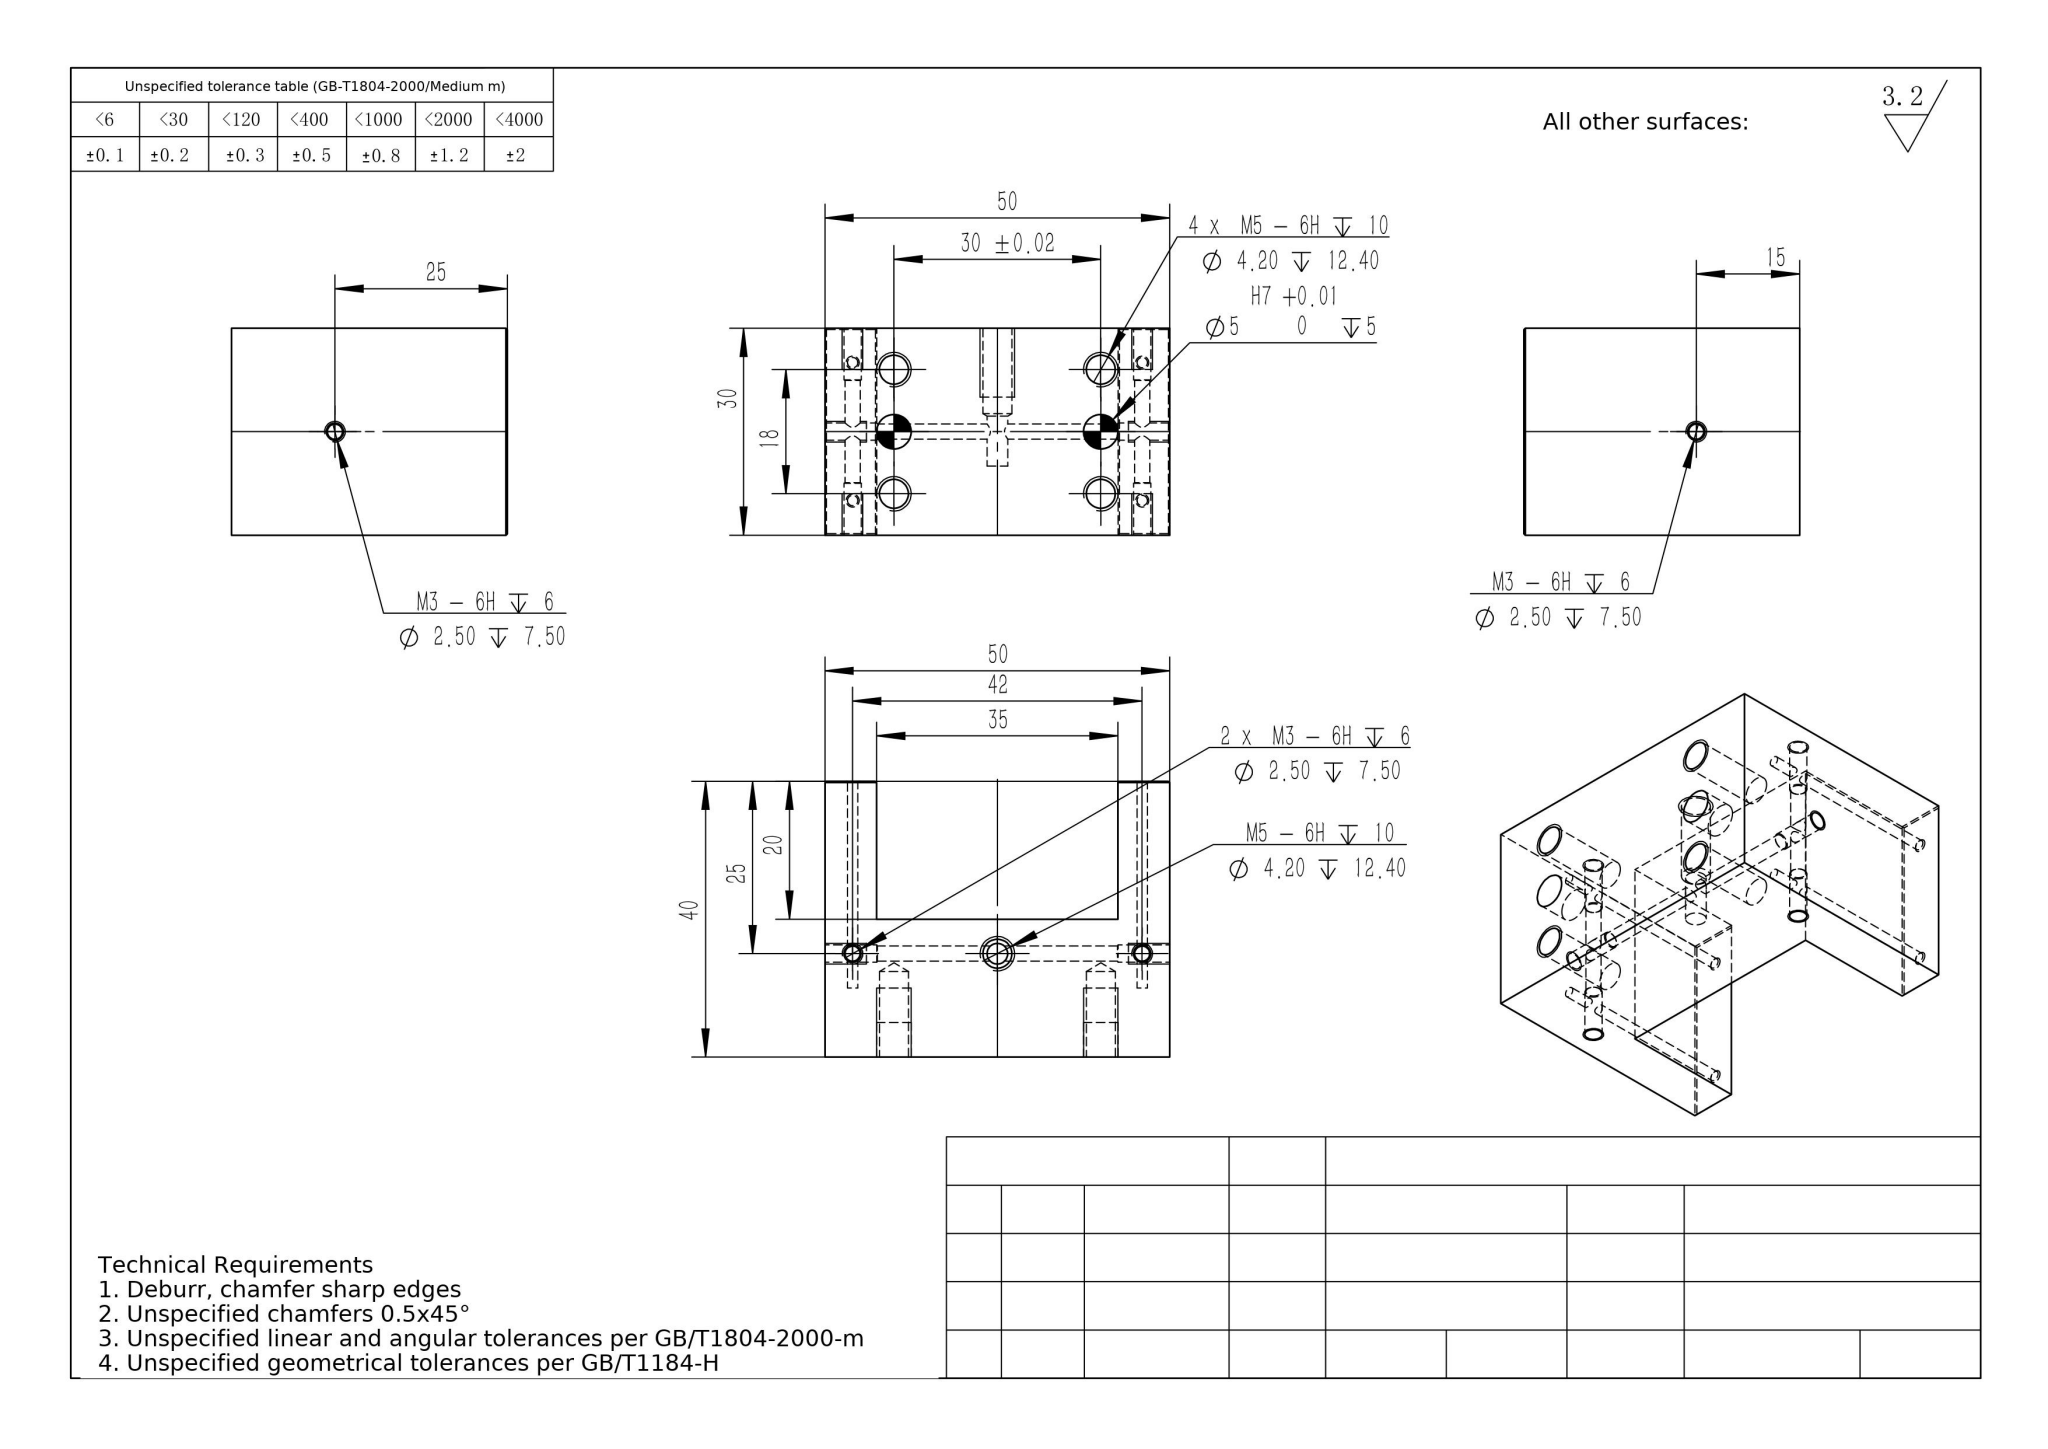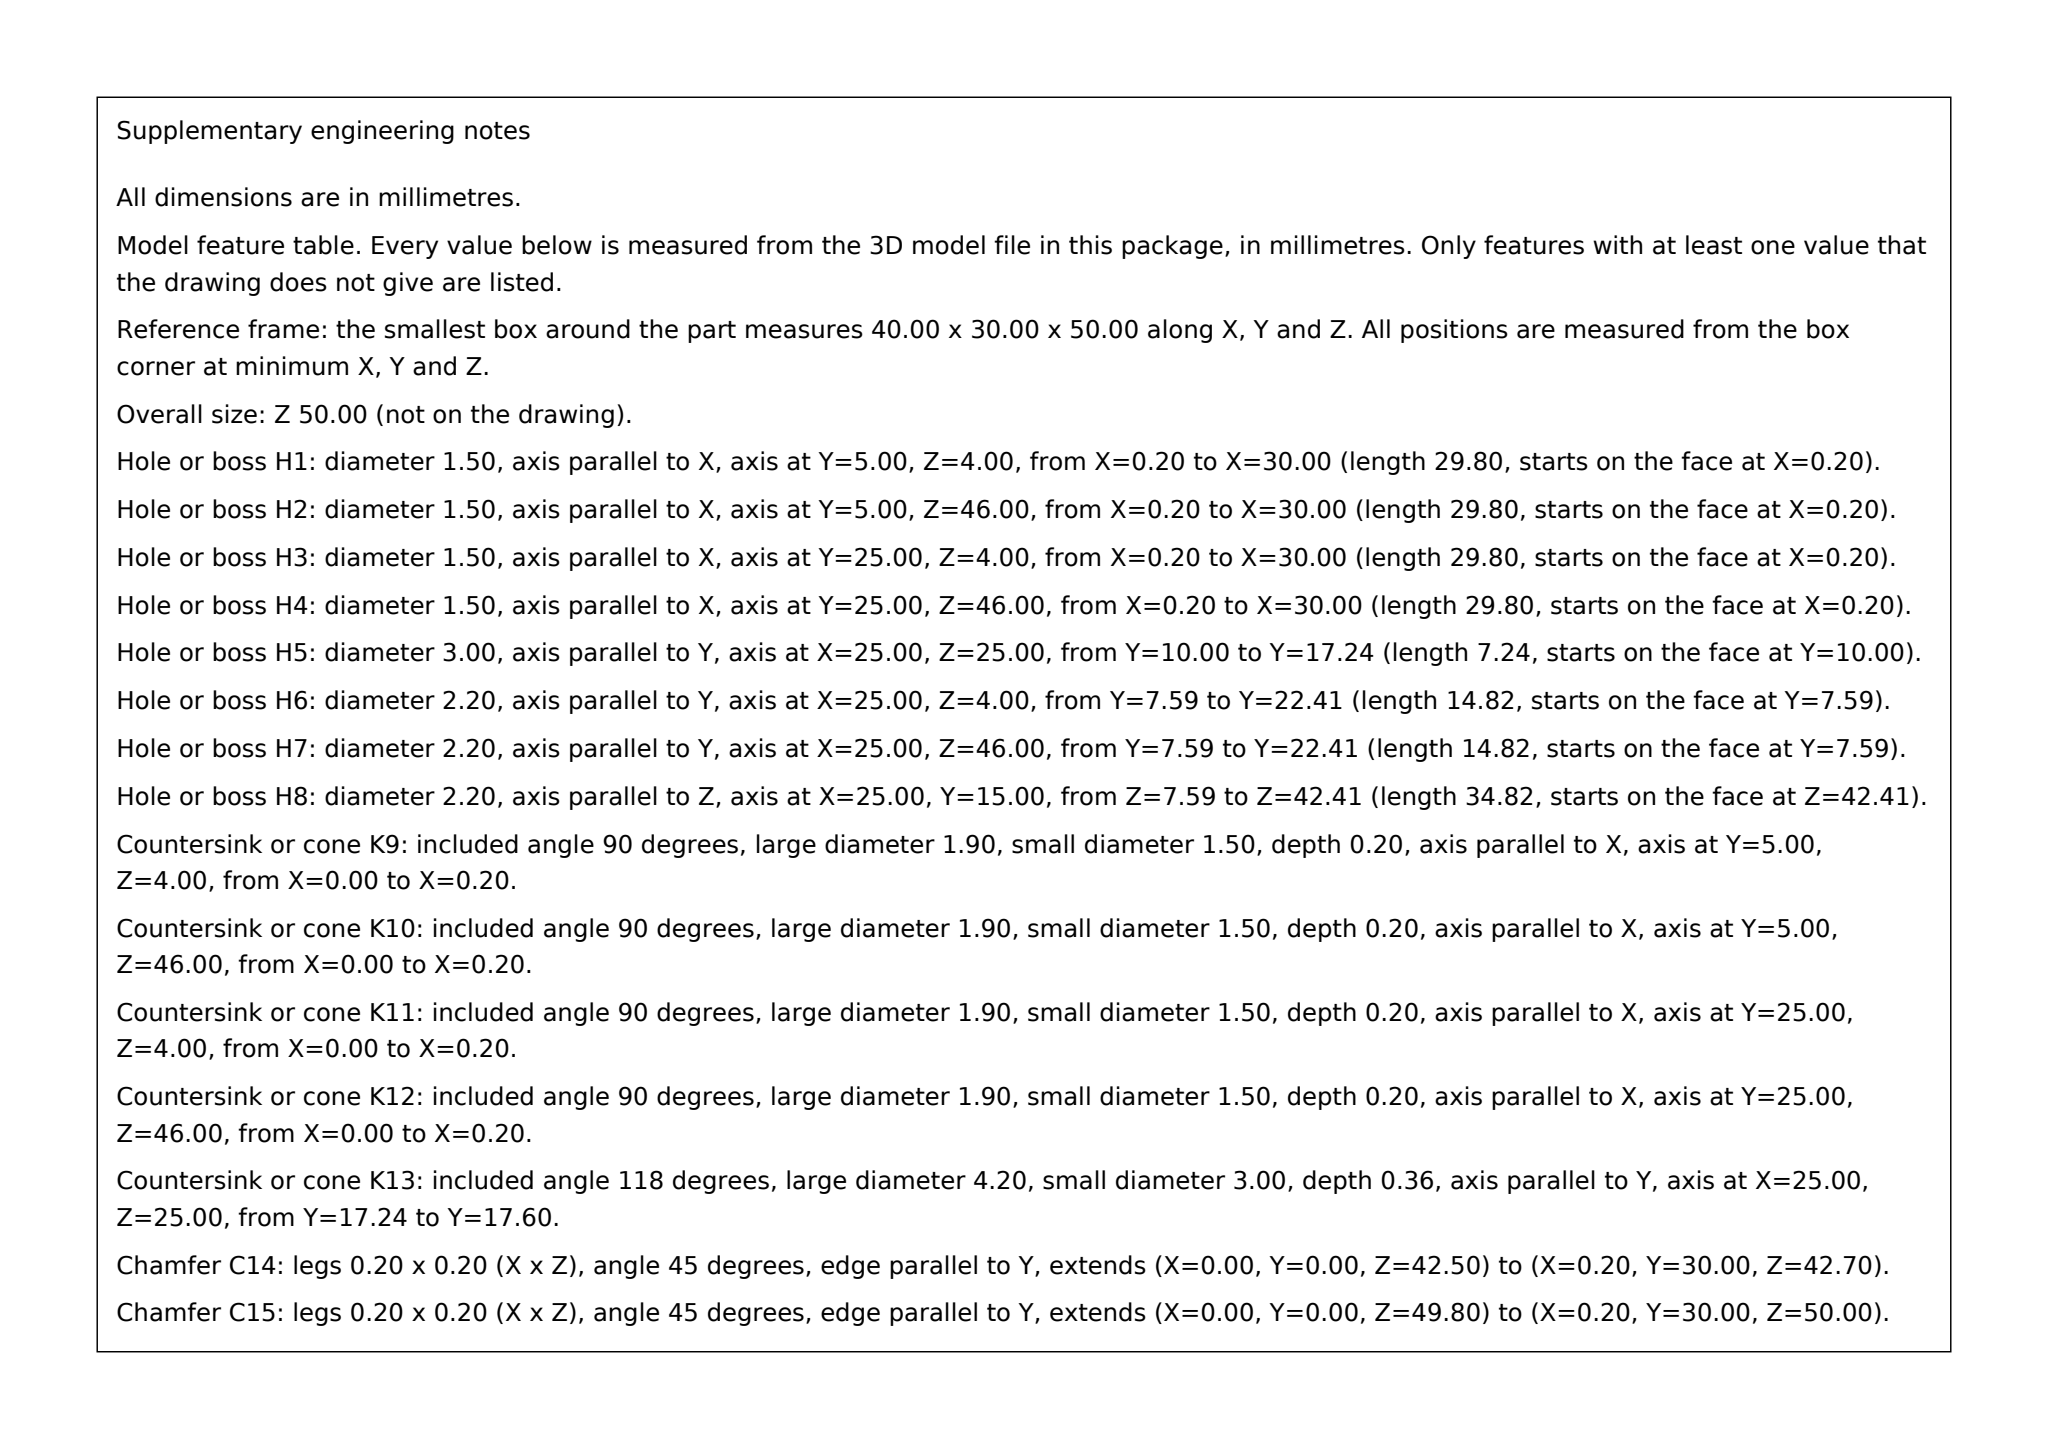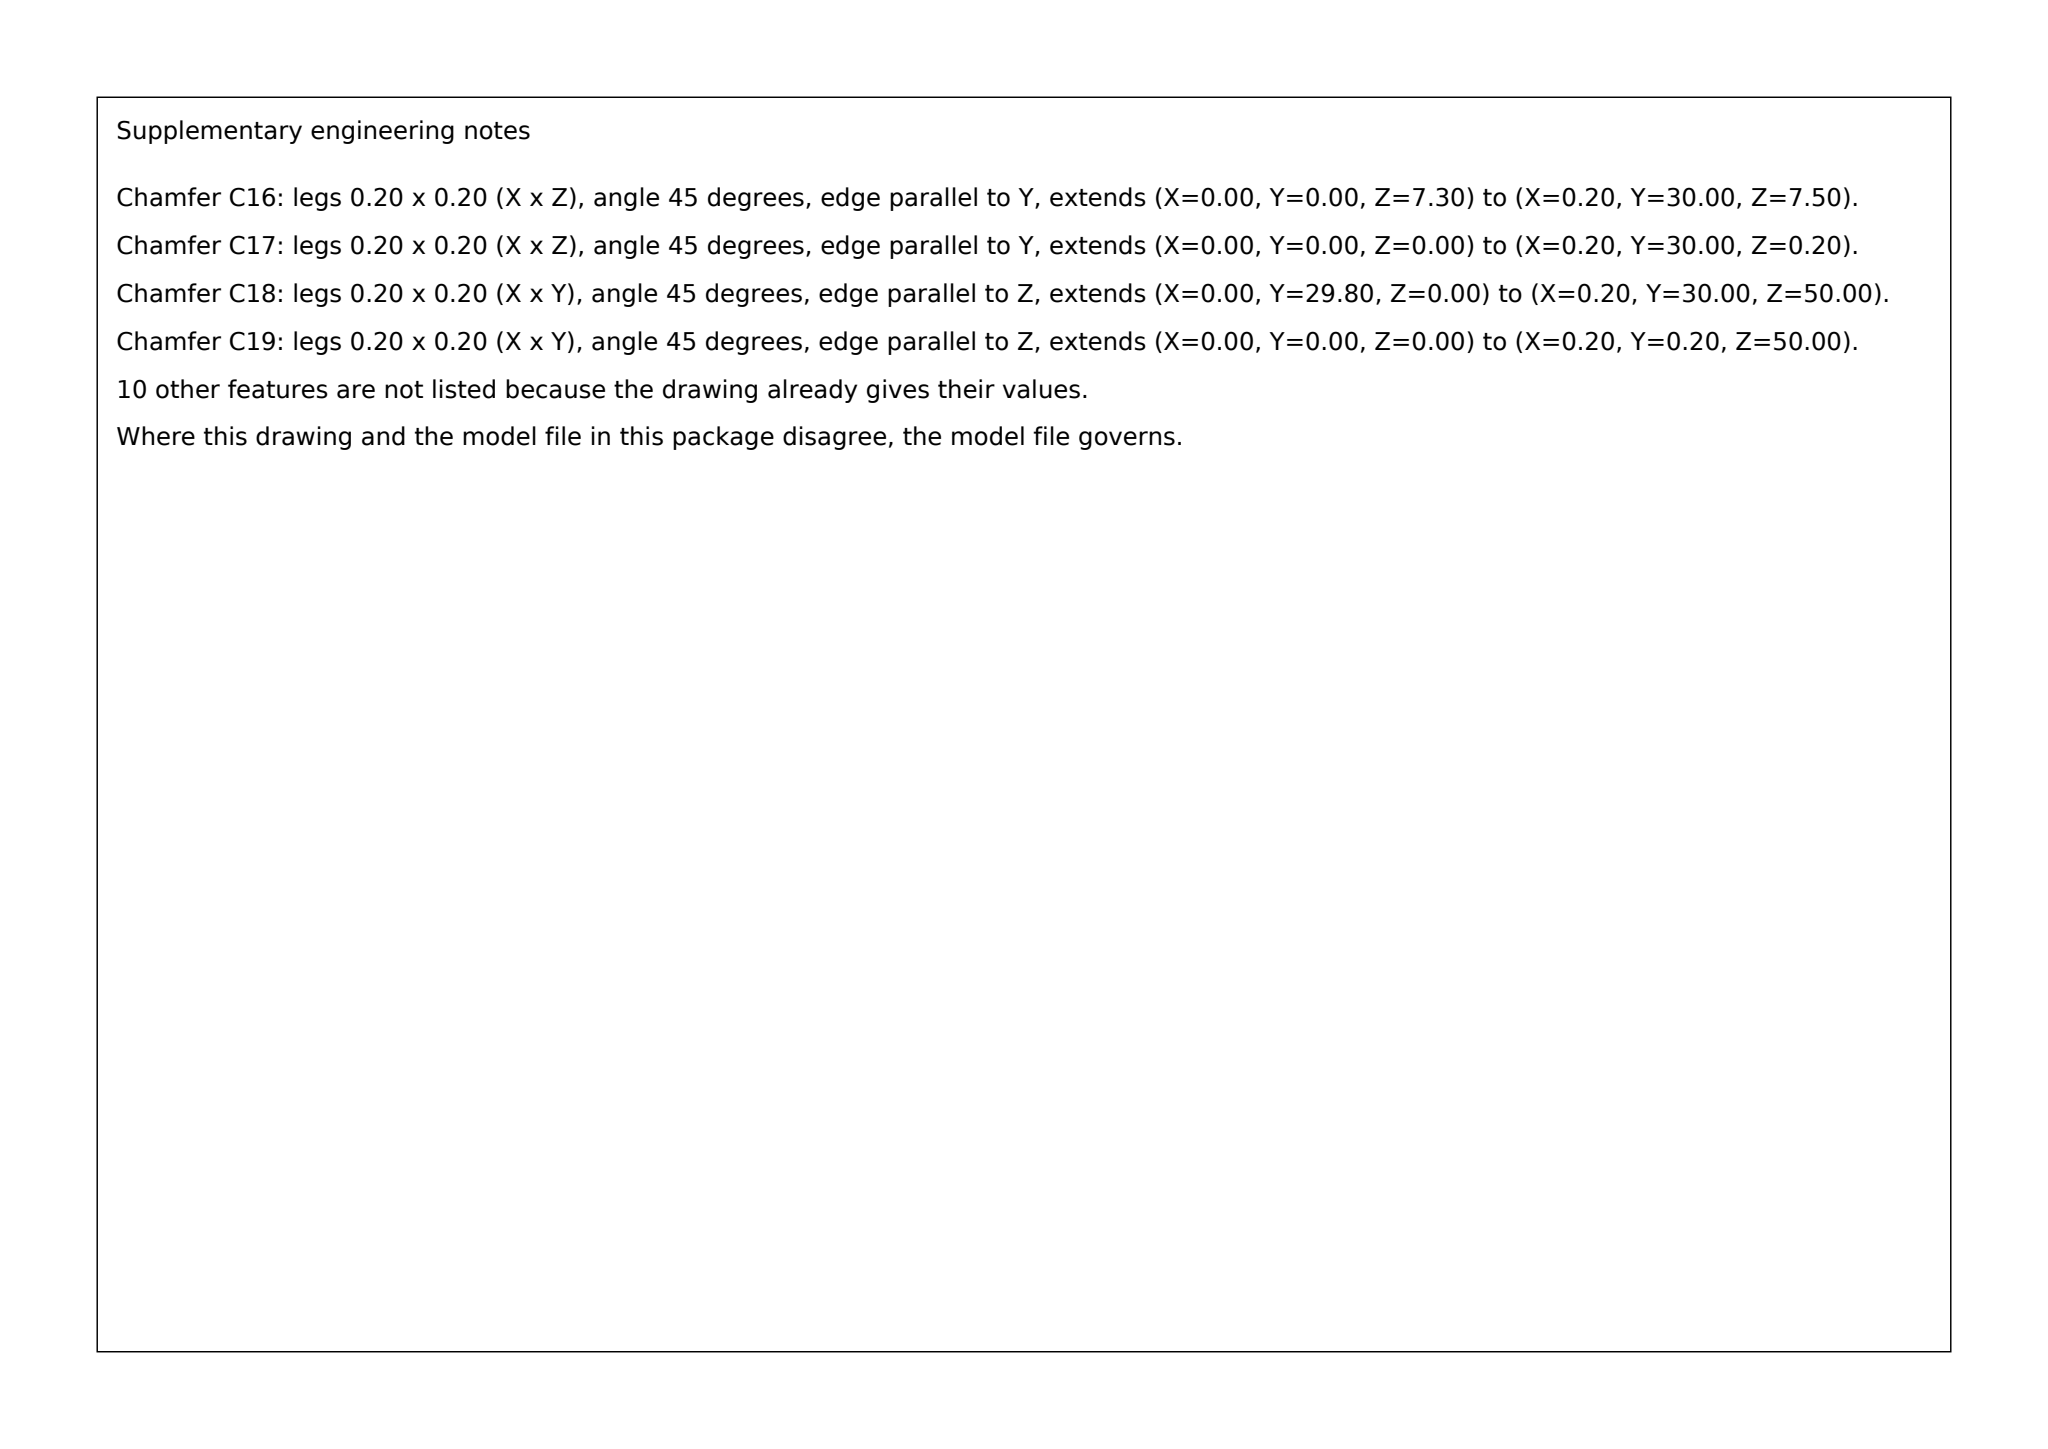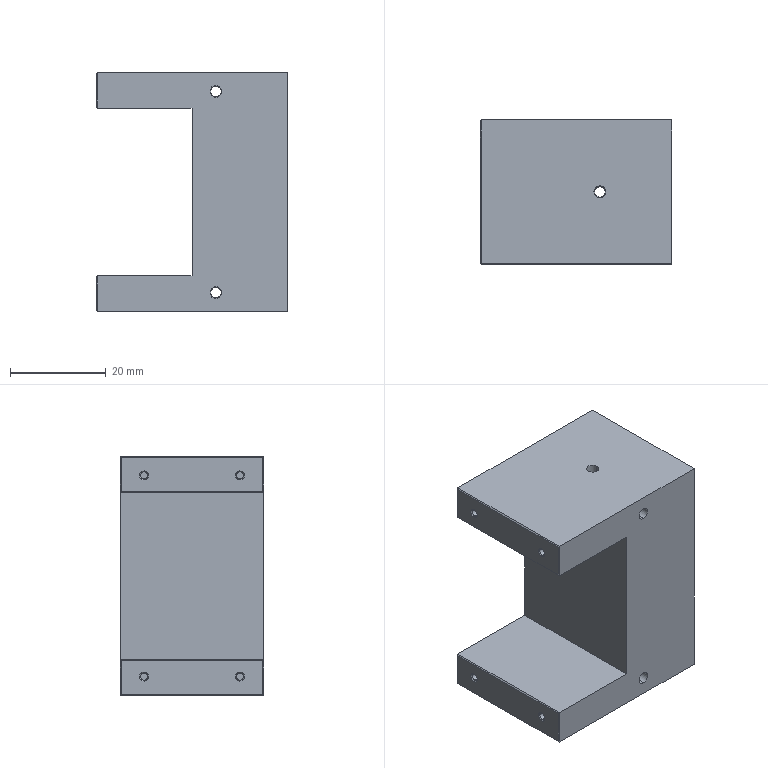Part | SolidWorks | mm | 1 solid | 111 faces | box 40 x 30 x 50 mm | volume 37227 mm3 | cylinder 56 | cone 30 | plane 25 | commonest cylinder face diameters 1.5 x16 2.5 x12 2.2 x12 4.2 x10 5 x4 3 x2
build123d program:
from build123d import *

# Parameters (mm, degrees)
SKETCH1_W             = 50
SKETCH1_H             = 30
BOSS_EXTRUDE1_DEPTH   = 40
SKETCH2_R             = 0.75
CUT_EXTRUDE1_DEPTH    = 30
SKETCH3_R             = 1.1
CUT_EXTRUDE2_DEPTH    = 56.902
SKETCH4_R             = 1.1
CUT_EXTRUDE3_DEPTH    = 66.765
SKETCH5_W             = 20
SKETCH5_H             = 35
CUT_EXTRUDE4_DEPTH    = 56.902
SKETCH6_R             = 1.5
CUT_EXTRUDE5_DEPTH    = 20
M3_TAPPED_HOLE3_D     = 2.5
M3_TAPPED_HOLE3_DEPTH = 7.5
M3_TAPPED_HOLE3_TIP   = 0.7511
M3_TAPPED_HOLE4_D     = 2.5
M3_TAPPED_HOLE4_DEPTH = 7.5
M3_TAPPED_HOLE4_TIP   = 0.7511
M3_TAPPED_HOLE2_D     = 2.5
M3_TAPPED_HOLE2_DEPTH = 7.5
M3_TAPPED_HOLE2_TIP   = 0.7511
M3_TAPPED_HOLE1_D     = 2.5
M3_TAPPED_HOLE1_DEPTH = 7.5
M3_TAPPED_HOLE1_TIP   = 0.7511
M5_TAPPED_HOLE5_D     = 4.2
M5_TAPPED_HOLE5_DEPTH = 12.4
M5_TAPPED_HOLE5_TIP   = 1.262
M5_TAPPED_HOLE6_D     = 4.2
M5_TAPPED_HOLE6_DEPTH = 12.4
M5_TAPPED_HOLE6_TIP   = 1.262
SKETCH20_R            = 2.5
CUT_EXTRUDE6_DEPTH    = 5
CHAMFER1_SIZE         = 0.2


with BuildPart() as part:
    # Sketch1 → Boss-Extrude1 (new body)
    with BuildSketch(Plane(origin=(0, 0, 0), x_dir=(0, 0, -1), z_dir=(1, 0, 0))):
        Rectangle(SKETCH1_W, SKETCH1_H)
    extrude(amount=BOSS_EXTRUDE1_DEPTH)

    # Sketch2 → Cut-Extrude1 (cut)
    with BuildSketch(Plane.ZY):
        with Locations((-21, 10)):
            Circle(SKETCH2_R)
        with Locations(Location((-21, -10, 0), (0, 0, 180))):
            Circle(SKETCH2_R)
        with Locations((21, -10)):
            Circle(SKETCH2_R)
        with Locations(Location((21, 10, 0), (0, 0, 180))):
            Circle(SKETCH2_R)
    extrude(amount=-CUT_EXTRUDE1_DEPTH, mode=Mode.SUBTRACT)

    # Sketch3 → Cut-Extrude2 (cut, through all)
    with BuildSketch(Plane(origin=(0, 15, 0), x_dir=(1, 0, 0), z_dir=(0, 1, 0))):
        with Locations(Location((25, 21, 0), (0, 0, 270))):
            Circle(SKETCH3_R)
        with Locations(Location((25, -21, 0), (0, 0, 90))):
            Circle(SKETCH3_R)
    extrude(amount=-CUT_EXTRUDE2_DEPTH, mode=Mode.SUBTRACT)

    # Sketch4 → Cut-Extrude3 (cut, through all)
    with BuildSketch(Plane.XY.offset(25)):
        with Locations((25, 0)):
            Circle(SKETCH4_R)
    extrude(amount=-CUT_EXTRUDE3_DEPTH, mode=Mode.SUBTRACT)

    # Sketch5 → Cut-Extrude4 (cut, through all)
    with BuildSketch(Plane(origin=(0, 15, 0), x_dir=(1, 0, 0), z_dir=(0, 1, 0))):
        with Locations((10, 0)):
            Rectangle(SKETCH5_W, SKETCH5_H)
    extrude(amount=-CUT_EXTRUDE4_DEPTH, mode=Mode.SUBTRACT)

    # Sketch6 → Cut-Extrude5 (cut)
    with BuildSketch(Plane(origin=(0, 15, 0), x_dir=(1, 0, 0), z_dir=(0, 1, 0))):
        with Locations(Location((25, 0, 0), (0, 0, 270))):
            Circle(SKETCH6_R)
    extrude(amount=-CUT_EXTRUDE5_DEPTH, mode=Mode.SUBTRACT)

    # M3 Tapped Hole3
    with Locations(Plane(origin=(0, 15, 0), x_dir=(1, 0, 0), z_dir=(0, 1, 0))):
        with Locations((25, 21), (25, -21)):
            Hole(M3_TAPPED_HOLE3_D / 2, depth=M3_TAPPED_HOLE3_DEPTH)
            with Locations((0, 0, -(M3_TAPPED_HOLE3_DEPTH + M3_TAPPED_HOLE3_TIP / 2))):  # 118° drill point
                Cone(0, M3_TAPPED_HOLE3_D / 2, M3_TAPPED_HOLE3_TIP, mode=Mode.SUBTRACT)

    # M3 Tapped Hole4
    with Locations(Plane(origin=(0, -15, 0), x_dir=(-1, 0, 0), z_dir=(0, -1, 0))):
        with Locations((-25, 21), (-25, -21)):
            Hole(M3_TAPPED_HOLE4_D / 2, depth=M3_TAPPED_HOLE4_DEPTH)
            with Locations((0, 0, -(M3_TAPPED_HOLE4_DEPTH + M3_TAPPED_HOLE4_TIP / 2))):  # 118° drill point
                Cone(0, M3_TAPPED_HOLE4_D / 2, M3_TAPPED_HOLE4_TIP, mode=Mode.SUBTRACT)

    # M3 Tapped Hole2
    with Locations(Plane(origin=(0, 0, -25), x_dir=(-1, 0, 0), z_dir=(0, 0, -1))):
        with Locations((-25, 0)):
            Hole(M3_TAPPED_HOLE2_D / 2, depth=M3_TAPPED_HOLE2_DEPTH)
            with Locations((0, 0, -(M3_TAPPED_HOLE2_DEPTH + M3_TAPPED_HOLE2_TIP / 2))):  # 118° drill point
                Cone(0, M3_TAPPED_HOLE2_D / 2, M3_TAPPED_HOLE2_TIP, mode=Mode.SUBTRACT)

    # M3 Tapped Hole1
    with Locations(Plane.XY.offset(25)):
        with Locations((25, 0)):
            Hole(M3_TAPPED_HOLE1_D / 2, depth=M3_TAPPED_HOLE1_DEPTH)
            with Locations((0, 0, -(M3_TAPPED_HOLE1_DEPTH + M3_TAPPED_HOLE1_TIP / 2))):  # 118° drill point
                Cone(0, M3_TAPPED_HOLE1_D / 2, M3_TAPPED_HOLE1_TIP, mode=Mode.SUBTRACT)

    # M5 Tapped Hole5
    with Locations(Plane(origin=(0, 15, 0), x_dir=(1, 0, 0), z_dir=(0, 1, 0))):
        with Locations((25, 0)):
            Hole(M5_TAPPED_HOLE5_D / 2, depth=M5_TAPPED_HOLE5_DEPTH)
            with Locations((0, 0, -(M5_TAPPED_HOLE5_DEPTH + M5_TAPPED_HOLE5_TIP / 2))):  # 118° drill point
                Cone(0, M5_TAPPED_HOLE5_D / 2, M5_TAPPED_HOLE5_TIP, mode=Mode.SUBTRACT)

    # M5 Tapped Hole6
    with Locations(Plane(origin=(40, 0, 0), x_dir=(0, 0, -1), z_dir=(1, 0, 0))):
        with Locations((-15, 9), (15, 9), (15, -9), (-15, -9)):
            Hole(M5_TAPPED_HOLE6_D / 2, depth=M5_TAPPED_HOLE6_DEPTH)
            with Locations((0, 0, -(M5_TAPPED_HOLE6_DEPTH + M5_TAPPED_HOLE6_TIP / 2))):  # 118° drill point
                Cone(0, M5_TAPPED_HOLE6_D / 2, M5_TAPPED_HOLE6_TIP, mode=Mode.SUBTRACT)

    # Sketch20 → Cut-Extrude6 (cut)
    with BuildSketch(Plane(origin=(40, 0, 0), x_dir=(0, 0, -1), z_dir=(1, 0, 0))):
        with Locations((15, 0)):
            Circle(SKETCH20_R)
        with Locations(Location((-15, 0, 0), (0, 0, 180))):
            Circle(SKETCH20_R)
    extrude(amount=-CUT_EXTRUDE6_DEPTH, mode=Mode.SUBTRACT)

    # Chamfer1
    chamfer1_edges = [part.edges().sort_by_distance(p)[0] for p in [
        (0, 10, 21.75),
        (0, -10, 20.25),
        (0, -10, -20.25),
        (0, 10, -21.75),
        (0, -15, 21.25),
        (0, 0, 25),
        (0, 15, -21.25),
        (0, 0, -25),
        (0, -15, -21.25),
        (0, 15, 21.25),
        (0, 0, 17.5),
        (0, 0, -17.5),
    ]]
    chamfer(chamfer1_edges, length=CHAMFER1_SIZE)


solid = part.part